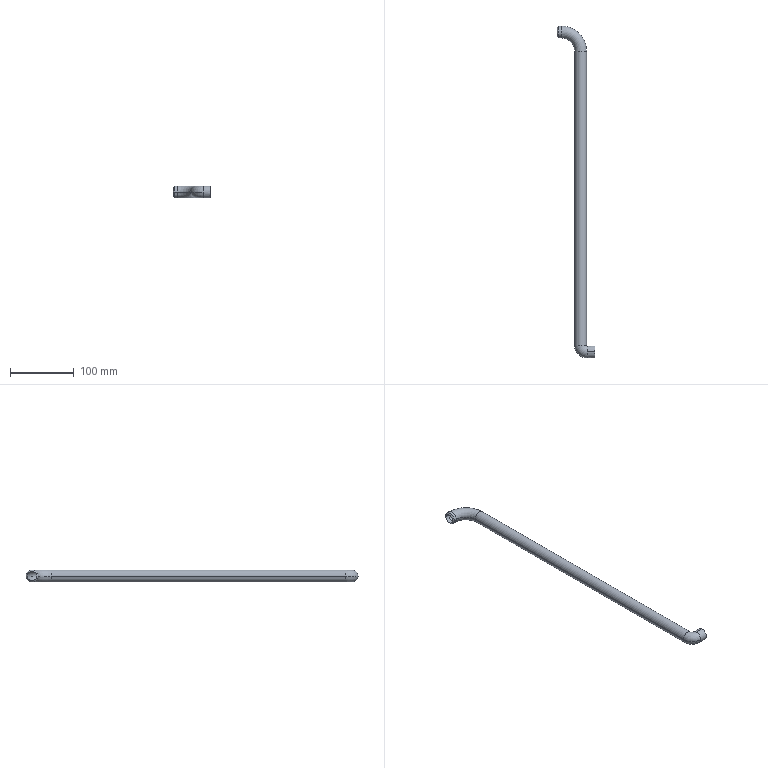Component | SolidWorks | PipeTwo-1 | 1 solid | 23 faces | box 59.27 x 519.6 x 18.77 mm | volume 54190 mm3 | cylinder 12 | torus 8 | cone 2 | plane 1 | commonest cylinder face diameters 15 x6 18.77 x6
STEP:
#1=COLOUR_RGB('',0.7922,0.8196,0.9333);
#2=FILL_AREA_STYLE_COLOUR('',#1);
#3=FILL_AREA_STYLE('',(#2));
#4=SURFACE_STYLE_FILL_AREA(#3);
#5=SURFACE_SIDE_STYLE('',(#4));
#6=SURFACE_STYLE_USAGE(.BOTH.,#5);
#7=PRESENTATION_STYLE_ASSIGNMENT((#6));
#8=CARTESIAN_POINT('',(24.858,12.574,4.921));
#9=VERTEX_POINT('',#8);
#10=CARTESIAN_POINT('',(25.448,12.574,4.921));
#11=VERTEX_POINT('',#10);
#12=CARTESIAN_POINT('',(25.153,12.574,4.921));
#13=DIRECTION('',(0.,-1.,0.));
#14=DIRECTION('',(0.,0.,1.));
#15=AXIS2_PLACEMENT_3D('',#12,#13,#14);
#16=CIRCLE('',#15,0.2953);
#17=EDGE_CURVE('',#9,#11,#16,.T.);
#18=ORIENTED_EDGE('',*,*,#17,.F.);
#19=CARTESIAN_POINT('',(25.547,11.885,4.921));
#20=VERTEX_POINT('',#19);
#21=CARTESIAN_POINT('',(25.547,12.574,4.921));
#22=DIRECTION('',(0.,0.,1.));
#23=DIRECTION('',(1.,0.,-0.));
#24=AXIS2_PLACEMENT_3D('',#21,#22,#23);
#25=CIRCLE('',#24,0.689);
#26=EDGE_CURVE('',#9,#20,#25,.T.);
#27=ORIENTED_EDGE('',*,*,#26,.T.);
#28=CARTESIAN_POINT('',(25.547,12.18,4.626));
#29=VERTEX_POINT('',#28);
#30=CARTESIAN_POINT('',(25.547,12.18,4.921));
#31=DIRECTION('',(1.,0.,-0.));
#32=DIRECTION('',(0.,0.,1.));
#33=AXIS2_PLACEMENT_3D('',#30,#31,#32);
#34=CIRCLE('',#33,0.2953);
#35=EDGE_CURVE('',#20,#29,#34,.T.);
#36=ORIENTED_EDGE('',*,*,#35,.T.);
#37=CARTESIAN_POINT('',(25.547,12.475,4.921));
#38=VERTEX_POINT('',#37);
#39=CARTESIAN_POINT('',(25.547,12.18,4.921));
#40=DIRECTION('',(1.,0.,-0.));
#41=DIRECTION('',(0.,0.,1.));
#42=AXIS2_PLACEMENT_3D('',#39,#40,#41);
#43=CIRCLE('',#42,0.2953);
#44=EDGE_CURVE('',#29,#38,#43,.T.);
#45=ORIENTED_EDGE('',*,*,#44,.T.);
#46=CARTESIAN_POINT('',(25.547,12.574,4.921));
#47=DIRECTION('',(0.,0.,1.));
#48=DIRECTION('',(1.,0.,0.));
#49=AXIS2_PLACEMENT_3D('',#46,#47,#48);
#50=CIRCLE('',#49,0.09843);
#51=EDGE_CURVE('',#11,#38,#50,.T.);
#52=ORIENTED_EDGE('',*,*,#51,.F.);
#53=EDGE_LOOP('',(#18,#27,#36,#45,#52));
#54=FACE_OUTER_BOUND('',#53,.T.);
#55=CARTESIAN_POINT('',(25.547,12.574,4.921));
#56=DIRECTION('',(0.,0.,1.));
#57=DIRECTION('',(1.,0.,-0.));
#58=AXIS2_PLACEMENT_3D('',#55,#56,#57);
#59=TOROIDAL_SURFACE('',#58,0.3937,0.2953);
#60=ADVANCED_FACE('',(#54),#59,.F.);
#61=CARTESIAN_POINT('',(23.972,32.193,4.921));
#62=VERTEX_POINT('',#61);
#63=CARTESIAN_POINT('',(23.972,31.602,4.921));
#64=VERTEX_POINT('',#63);
#65=CARTESIAN_POINT('',(23.972,31.898,4.921));
#66=DIRECTION('',(1.,0.,-0.));
#67=DIRECTION('',(0.,0.,1.));
#68=AXIS2_PLACEMENT_3D('',#65,#66,#67);
#69=CIRCLE('',#68,0.2953);
#70=EDGE_CURVE('',#62,#64,#69,.T.);
#71=ORIENTED_EDGE('',*,*,#70,.F.);
#72=CARTESIAN_POINT('',(25.448,30.717,4.921));
#73=VERTEX_POINT('',#72);
#74=CARTESIAN_POINT('',(23.972,30.717,4.921));
#75=DIRECTION('',(-0.,-0.,-1.));
#76=DIRECTION('',(-1.,0.,0.));
#77=AXIS2_PLACEMENT_3D('',#74,#75,#76);
#78=CIRCLE('',#77,1.476);
#79=EDGE_CURVE('',#62,#73,#78,.T.);
#80=ORIENTED_EDGE('',*,*,#79,.T.);
#81=CARTESIAN_POINT('',(24.858,30.717,4.921));
#82=VERTEX_POINT('',#81);
#83=CARTESIAN_POINT('',(25.153,30.717,4.921));
#84=DIRECTION('',(0.,-1.,0.));
#85=DIRECTION('',(0.,0.,1.));
#86=AXIS2_PLACEMENT_3D('',#83,#84,#85);
#87=CIRCLE('',#86,0.2953);
#88=EDGE_CURVE('',#73,#82,#87,.T.);
#89=ORIENTED_EDGE('',*,*,#88,.T.);
#90=CARTESIAN_POINT('',(23.972,30.717,4.921));
#91=DIRECTION('',(-0.,-0.,-1.));
#92=DIRECTION('',(-1.,0.,0.));
#93=AXIS2_PLACEMENT_3D('',#90,#91,#92);
#94=CIRCLE('',#93,0.8858);
#95=EDGE_CURVE('',#64,#82,#94,.T.);
#96=ORIENTED_EDGE('',*,*,#95,.F.);
#97=EDGE_LOOP('',(#71,#80,#89,#96));
#98=FACE_OUTER_BOUND('',#97,.T.);
#99=CARTESIAN_POINT('',(23.972,30.717,4.921));
#100=DIRECTION('',(-0.,-0.,-1.));
#101=DIRECTION('',(-1.,-0.,0.));
#102=AXIS2_PLACEMENT_3D('',#99,#100,#101);
#103=TOROIDAL_SURFACE('',#102,1.181,0.2953);
#104=ADVANCED_FACE('',(#98),#103,.F.);
#105=CARTESIAN_POINT('',(24.784,12.574,4.921));
#106=VERTEX_POINT('',#105);
#107=CARTESIAN_POINT('',(25.523,12.574,4.921));
#108=VERTEX_POINT('',#107);
#109=CARTESIAN_POINT('',(25.153,12.574,4.921));
#110=DIRECTION('',(-0.,1.,-0.));
#111=DIRECTION('',(0.,0.,1.));
#112=AXIS2_PLACEMENT_3D('',#109,#110,#111);
#113=CIRCLE('',#112,0.3695);
#114=EDGE_CURVE('',#106,#108,#113,.T.);
#115=ORIENTED_EDGE('',*,*,#114,.F.);
#116=CARTESIAN_POINT('',(25.547,11.81,4.921));
#117=VERTEX_POINT('',#116);
#118=CARTESIAN_POINT('',(25.547,12.574,4.921));
#119=DIRECTION('',(0.,0.,1.));
#120=DIRECTION('',(1.,0.,-0.));
#121=AXIS2_PLACEMENT_3D('',#118,#119,#120);
#122=CIRCLE('',#121,0.7632);
#123=EDGE_CURVE('',#106,#117,#122,.T.);
#124=ORIENTED_EDGE('',*,*,#123,.T.);
#125=CARTESIAN_POINT('',(25.547,12.18,5.291));
#126=VERTEX_POINT('',#125);
#127=CARTESIAN_POINT('',(25.547,12.18,4.921));
#128=DIRECTION('',(-1.,-0.,0.));
#129=DIRECTION('',(0.,0.,1.));
#130=AXIS2_PLACEMENT_3D('',#127,#128,#129);
#131=CIRCLE('',#130,0.3695);
#132=EDGE_CURVE('',#117,#126,#131,.T.);
#133=ORIENTED_EDGE('',*,*,#132,.T.);
#134=CARTESIAN_POINT('',(25.547,12.549,4.921));
#135=VERTEX_POINT('',#134);
#136=CARTESIAN_POINT('',(25.547,12.18,4.921));
#137=DIRECTION('',(-1.,-0.,0.));
#138=DIRECTION('',(0.,0.,1.));
#139=AXIS2_PLACEMENT_3D('',#136,#137,#138);
#140=CIRCLE('',#139,0.3695);
#141=EDGE_CURVE('',#126,#135,#140,.T.);
#142=ORIENTED_EDGE('',*,*,#141,.T.);
#143=CARTESIAN_POINT('',(25.547,12.574,4.921));
#144=DIRECTION('',(0.,0.,1.));
#145=DIRECTION('',(1.,0.,0.));
#146=AXIS2_PLACEMENT_3D('',#143,#144,#145);
#147=CIRCLE('',#146,0.02421);
#148=EDGE_CURVE('',#108,#135,#147,.T.);
#149=ORIENTED_EDGE('',*,*,#148,.F.);
#150=EDGE_LOOP('',(#115,#124,#133,#142,#149));
#151=FACE_OUTER_BOUND('',#150,.T.);
#152=CARTESIAN_POINT('',(25.547,12.574,4.921));
#153=DIRECTION('',(0.,0.,1.));
#154=DIRECTION('',(1.,0.,-0.));
#155=AXIS2_PLACEMENT_3D('',#152,#153,#154);
#156=TOROIDAL_SURFACE('',#155,0.3937,0.3695);
#157=ADVANCED_FACE('',(#151),#156,.T.);
#158=CARTESIAN_POINT('',(23.972,32.267,4.921));
#159=VERTEX_POINT('',#158);
#160=CARTESIAN_POINT('',(23.972,31.528,4.921));
#161=VERTEX_POINT('',#160);
#162=CARTESIAN_POINT('',(23.972,31.898,4.921));
#163=DIRECTION('',(-1.,-0.,0.));
#164=DIRECTION('',(0.,0.,1.));
#165=AXIS2_PLACEMENT_3D('',#162,#163,#164);
#166=CIRCLE('',#165,0.3695);
#167=EDGE_CURVE('',#159,#161,#166,.T.);
#168=ORIENTED_EDGE('',*,*,#167,.F.);
#169=CARTESIAN_POINT('',(25.523,30.717,4.921));
#170=VERTEX_POINT('',#169);
#171=CARTESIAN_POINT('',(23.972,30.717,4.921));
#172=DIRECTION('',(-0.,-0.,-1.));
#173=DIRECTION('',(-1.,0.,0.));
#174=AXIS2_PLACEMENT_3D('',#171,#172,#173);
#175=CIRCLE('',#174,1.551);
#176=EDGE_CURVE('',#159,#170,#175,.T.);
#177=ORIENTED_EDGE('',*,*,#176,.T.);
#178=CARTESIAN_POINT('',(24.784,30.717,4.921));
#179=VERTEX_POINT('',#178);
#180=CARTESIAN_POINT('',(25.153,30.717,4.921));
#181=DIRECTION('',(-0.,1.,-0.));
#182=DIRECTION('',(0.,0.,1.));
#183=AXIS2_PLACEMENT_3D('',#180,#181,#182);
#184=CIRCLE('',#183,0.3695);
#185=EDGE_CURVE('',#170,#179,#184,.T.);
#186=ORIENTED_EDGE('',*,*,#185,.T.);
#187=CARTESIAN_POINT('',(23.972,30.717,4.921));
#188=DIRECTION('',(-0.,-0.,-1.));
#189=DIRECTION('',(-1.,0.,0.));
#190=AXIS2_PLACEMENT_3D('',#187,#188,#189);
#191=CIRCLE('',#190,0.8116);
#192=EDGE_CURVE('',#161,#179,#191,.T.);
#193=ORIENTED_EDGE('',*,*,#192,.F.);
#194=EDGE_LOOP('',(#168,#177,#186,#193));
#195=FACE_OUTER_BOUND('',#194,.T.);
#196=CARTESIAN_POINT('',(23.972,30.717,4.921));
#197=DIRECTION('',(-0.,-0.,-1.));
#198=DIRECTION('',(-1.,-0.,0.));
#199=AXIS2_PLACEMENT_3D('',#196,#197,#198);
#200=TOROIDAL_SURFACE('',#199,1.181,0.3695);
#201=ADVANCED_FACE('',(#195),#200,.T.);
#202=CARTESIAN_POINT('',(23.701,32.193,4.921));
#203=VERTEX_POINT('',#202);
#204=CARTESIAN_POINT('',(23.701,31.602,4.921));
#205=VERTEX_POINT('',#204);
#206=CARTESIAN_POINT('',(23.701,31.898,4.921));
#207=DIRECTION('',(-1.,-0.,0.));
#208=DIRECTION('',(0.,-1.,0.));
#209=AXIS2_PLACEMENT_3D('',#206,#207,#208);
#210=CIRCLE('',#209,0.2953);
#211=EDGE_CURVE('',#203,#205,#210,.T.);
#212=ORIENTED_EDGE('',*,*,#211,.F.);
#213=CARTESIAN_POINT('',(23.775,32.267,4.921));
#214=VERTEX_POINT('',#213);
#215=CARTESIAN_POINT('',(23.578,32.07,4.921));
#216=DIRECTION('',(0.7071,0.7071,-0.));
#217=VECTOR('',#216,39.37);
#218=LINE('',#215,#217);
#219=EDGE_CURVE('',#203,#214,#218,.T.);
#220=ORIENTED_EDGE('',*,*,#219,.T.);
#221=CARTESIAN_POINT('',(23.775,31.528,4.921));
#222=VERTEX_POINT('',#221);
#223=CARTESIAN_POINT('',(23.775,31.898,4.921));
#224=DIRECTION('',(1.,0.,-0.));
#225=DIRECTION('',(0.,1.,0.));
#226=AXIS2_PLACEMENT_3D('',#223,#224,#225);
#227=CIRCLE('',#226,0.3695);
#228=EDGE_CURVE('',#222,#214,#227,.T.);
#229=ORIENTED_EDGE('',*,*,#228,.F.);
#230=CARTESIAN_POINT('',(23.578,31.725,4.921));
#231=DIRECTION('',(0.7071,-0.7071,-0.));
#232=VECTOR('',#231,39.37);
#233=LINE('',#230,#232);
#234=EDGE_CURVE('',#205,#222,#233,.T.);
#235=ORIENTED_EDGE('',*,*,#234,.F.);
#236=EDGE_LOOP('',(#212,#220,#229,#235));
#237=FACE_OUTER_BOUND('',#236,.T.);
#238=CARTESIAN_POINT('',(23.578,31.898,4.921));
#239=DIRECTION('',(1.,0.,-0.));
#240=DIRECTION('',(0.,-1.,0.));
#241=AXIS2_PLACEMENT_3D('',#238,#239,#240);
#242=CONICAL_SURFACE('',#241,0.1726,0.7854);
#243=ADVANCED_FACE('',(#237),#242,.T.);
#244=CARTESIAN_POINT('',(25.547,12.18,5.217));
#245=VERTEX_POINT('',#244);
#246=CARTESIAN_POINT('',(25.547,12.18,4.921));
#247=DIRECTION('',(1.,0.,-0.));
#248=DIRECTION('',(0.,0.,1.));
#249=AXIS2_PLACEMENT_3D('',#246,#247,#248);
#250=CIRCLE('',#249,0.2953);
#251=EDGE_CURVE('',#245,#20,#250,.T.);
#252=ORIENTED_EDGE('',*,*,#251,.F.);
#253=CARTESIAN_POINT('',(26.034,12.18,5.217));
#254=VERTEX_POINT('',#253);
#255=CARTESIAN_POINT('',(25.547,12.18,5.217));
#256=DIRECTION('',(1.,0.,-0.));
#257=VECTOR('',#256,39.37);
#258=LINE('',#255,#257);
#259=EDGE_CURVE('',#245,#254,#258,.T.);
#260=ORIENTED_EDGE('',*,*,#259,.T.);
#261=CARTESIAN_POINT('',(26.034,12.18,4.626));
#262=VERTEX_POINT('',#261);
#263=CARTESIAN_POINT('',(26.034,12.18,4.921));
#264=DIRECTION('',(1.,0.,-0.));
#265=DIRECTION('',(0.,0.,1.));
#266=AXIS2_PLACEMENT_3D('',#263,#264,#265);
#267=CIRCLE('',#266,0.2953);
#268=EDGE_CURVE('',#254,#262,#267,.T.);
#269=ORIENTED_EDGE('',*,*,#268,.T.);
#270=CARTESIAN_POINT('',(25.547,12.18,4.626));
#271=DIRECTION('',(1.,0.,-0.));
#272=VECTOR('',#271,39.37);
#273=LINE('',#270,#272);
#274=EDGE_CURVE('',#29,#262,#273,.T.);
#275=ORIENTED_EDGE('',*,*,#274,.F.);
#276=ORIENTED_EDGE('',*,*,#35,.F.);
#277=EDGE_LOOP('',(#252,#260,#269,#275,#276));
#278=FACE_OUTER_BOUND('',#277,.T.);
#279=CARTESIAN_POINT('',(25.547,12.18,4.921));
#280=DIRECTION('',(1.,0.,-0.));
#281=DIRECTION('',(0.,0.,-1.));
#282=AXIS2_PLACEMENT_3D('',#279,#280,#281);
#283=CYLINDRICAL_SURFACE('',#282,0.2953);
#284=ADVANCED_FACE('',(#278),#283,.F.);
#285=ORIENTED_EDGE('',*,*,#88,.F.);
#286=CARTESIAN_POINT('',(25.448,30.717,4.921));
#287=DIRECTION('',(0.,-1.,0.));
#288=VECTOR('',#287,39.37);
#289=LINE('',#286,#288);
#290=EDGE_CURVE('',#73,#11,#289,.T.);
#291=ORIENTED_EDGE('',*,*,#290,.T.);
#292=CARTESIAN_POINT('',(25.153,12.574,4.921));
#293=DIRECTION('',(0.,-1.,0.));
#294=DIRECTION('',(0.,0.,1.));
#295=AXIS2_PLACEMENT_3D('',#292,#293,#294);
#296=CIRCLE('',#295,0.2953);
#297=EDGE_CURVE('',#11,#9,#296,.T.);
#298=ORIENTED_EDGE('',*,*,#297,.T.);
#299=CARTESIAN_POINT('',(24.858,30.717,4.921));
#300=DIRECTION('',(0.,-1.,0.));
#301=VECTOR('',#300,39.37);
#302=LINE('',#299,#301);
#303=EDGE_CURVE('',#82,#9,#302,.T.);
#304=ORIENTED_EDGE('',*,*,#303,.F.);
#305=EDGE_LOOP('',(#285,#291,#298,#304));
#306=FACE_OUTER_BOUND('',#305,.T.);
#307=CARTESIAN_POINT('',(25.153,30.717,4.921));
#308=DIRECTION('',(0.,-1.,0.));
#309=DIRECTION('',(-1.,0.,0.));
#310=AXIS2_PLACEMENT_3D('',#307,#308,#309);
#311=CYLINDRICAL_SURFACE('',#310,0.2953);
#312=ADVANCED_FACE('',(#306),#311,.F.);
#313=CARTESIAN_POINT('',(23.701,31.898,4.921));
#314=DIRECTION('',(-1.,-0.,0.));
#315=DIRECTION('',(0.,-1.,0.));
#316=AXIS2_PLACEMENT_3D('',#313,#314,#315);
#317=CIRCLE('',#316,0.2953);
#318=EDGE_CURVE('',#205,#203,#317,.T.);
#319=ORIENTED_EDGE('',*,*,#318,.T.);
#320=CARTESIAN_POINT('',(23.578,32.193,4.921));
#321=DIRECTION('',(1.,0.,-0.));
#322=VECTOR('',#321,39.37);
#323=LINE('',#320,#322);
#324=EDGE_CURVE('',#203,#62,#323,.T.);
#325=ORIENTED_EDGE('',*,*,#324,.T.);
#326=ORIENTED_EDGE('',*,*,#70,.T.);
#327=CARTESIAN_POINT('',(23.578,31.602,4.921));
#328=DIRECTION('',(1.,0.,-0.));
#329=VECTOR('',#328,39.37);
#330=LINE('',#327,#329);
#331=EDGE_CURVE('',#205,#64,#330,.T.);
#332=ORIENTED_EDGE('',*,*,#331,.F.);
#333=EDGE_LOOP('',(#319,#325,#326,#332));
#334=FACE_OUTER_BOUND('',#333,.T.);
#335=CARTESIAN_POINT('',(23.578,31.898,4.921));
#336=DIRECTION('',(1.,0.,-0.));
#337=DIRECTION('',(0.,-1.,0.));
#338=AXIS2_PLACEMENT_3D('',#335,#336,#337);
#339=CYLINDRICAL_SURFACE('',#338,0.2953);
#340=ADVANCED_FACE('',(#334),#339,.F.);
#341=ORIENTED_EDGE('',*,*,#141,.F.);
#342=CARTESIAN_POINT('',(26.034,12.18,5.291));
#343=VERTEX_POINT('',#342);
#344=CARTESIAN_POINT('',(25.547,12.18,5.291));
#345=DIRECTION('',(1.,0.,-0.));
#346=VECTOR('',#345,39.37);
#347=LINE('',#344,#346);
#348=EDGE_CURVE('',#126,#343,#347,.T.);
#349=ORIENTED_EDGE('',*,*,#348,.T.);
#350=CARTESIAN_POINT('',(26.034,12.18,4.552));
#351=VERTEX_POINT('',#350);
#352=CARTESIAN_POINT('',(26.034,12.18,4.921));
#353=DIRECTION('',(-1.,-0.,0.));
#354=DIRECTION('',(0.,0.,1.));
#355=AXIS2_PLACEMENT_3D('',#352,#353,#354);
#356=CIRCLE('',#355,0.3695);
#357=EDGE_CURVE('',#343,#351,#356,.T.);
#358=ORIENTED_EDGE('',*,*,#357,.T.);
#359=CARTESIAN_POINT('',(25.547,12.18,4.552));
#360=VERTEX_POINT('',#359);
#361=CARTESIAN_POINT('',(25.547,12.18,4.552));
#362=DIRECTION('',(1.,0.,-0.));
#363=VECTOR('',#362,39.37);
#364=LINE('',#361,#363);
#365=EDGE_CURVE('',#360,#351,#364,.T.);
#366=ORIENTED_EDGE('',*,*,#365,.F.);
#367=CARTESIAN_POINT('',(25.547,12.18,4.921));
#368=DIRECTION('',(-1.,-0.,0.));
#369=DIRECTION('',(0.,0.,1.));
#370=AXIS2_PLACEMENT_3D('',#367,#368,#369);
#371=CIRCLE('',#370,0.3695);
#372=EDGE_CURVE('',#135,#360,#371,.T.);
#373=ORIENTED_EDGE('',*,*,#372,.F.);
#374=EDGE_LOOP('',(#341,#349,#358,#366,#373));
#375=FACE_OUTER_BOUND('',#374,.T.);
#376=CARTESIAN_POINT('',(25.547,12.18,4.921));
#377=DIRECTION('',(1.,0.,-0.));
#378=DIRECTION('',(0.,0.,-1.));
#379=AXIS2_PLACEMENT_3D('',#376,#377,#378);
#380=CYLINDRICAL_SURFACE('',#379,0.3695);
#381=ADVANCED_FACE('',(#375),#380,.T.);
#382=ORIENTED_EDGE('',*,*,#185,.F.);
#383=CARTESIAN_POINT('',(25.523,30.717,4.921));
#384=DIRECTION('',(0.,-1.,0.));
#385=VECTOR('',#384,39.37);
#386=LINE('',#383,#385);
#387=EDGE_CURVE('',#170,#108,#386,.T.);
#388=ORIENTED_EDGE('',*,*,#387,.T.);
#389=CARTESIAN_POINT('',(25.153,12.574,4.921));
#390=DIRECTION('',(-0.,1.,-0.));
#391=DIRECTION('',(0.,0.,1.));
#392=AXIS2_PLACEMENT_3D('',#389,#390,#391);
#393=CIRCLE('',#392,0.3695);
#394=EDGE_CURVE('',#108,#106,#393,.T.);
#395=ORIENTED_EDGE('',*,*,#394,.T.);
#396=CARTESIAN_POINT('',(24.784,30.717,4.921));
#397=DIRECTION('',(0.,-1.,0.));
#398=VECTOR('',#397,39.37);
#399=LINE('',#396,#398);
#400=EDGE_CURVE('',#179,#106,#399,.T.);
#401=ORIENTED_EDGE('',*,*,#400,.F.);
#402=EDGE_LOOP('',(#382,#388,#395,#401));
#403=FACE_OUTER_BOUND('',#402,.T.);
#404=CARTESIAN_POINT('',(25.153,30.717,4.921));
#405=DIRECTION('',(0.,-1.,0.));
#406=DIRECTION('',(-1.,0.,0.));
#407=AXIS2_PLACEMENT_3D('',#404,#405,#406);
#408=CYLINDRICAL_SURFACE('',#407,0.3695);
#409=ADVANCED_FACE('',(#403),#408,.T.);
#410=ORIENTED_EDGE('',*,*,#228,.T.);
#411=CARTESIAN_POINT('',(23.578,32.267,4.921));
#412=DIRECTION('',(1.,0.,-0.));
#413=VECTOR('',#412,39.37);
#414=LINE('',#411,#413);
#415=EDGE_CURVE('',#214,#159,#414,.T.);
#416=ORIENTED_EDGE('',*,*,#415,.T.);
#417=ORIENTED_EDGE('',*,*,#167,.T.);
#418=CARTESIAN_POINT('',(23.578,31.528,4.921));
#419=DIRECTION('',(1.,0.,-0.));
#420=VECTOR('',#419,39.37);
#421=LINE('',#418,#420);
#422=EDGE_CURVE('',#222,#161,#421,.T.);
#423=ORIENTED_EDGE('',*,*,#422,.F.);
#424=EDGE_LOOP('',(#410,#416,#417,#423));
#425=FACE_OUTER_BOUND('',#424,.T.);
#426=CARTESIAN_POINT('',(23.578,31.898,4.921));
#427=DIRECTION('',(1.,0.,-0.));
#428=DIRECTION('',(0.,-1.,0.));
#429=AXIS2_PLACEMENT_3D('',#426,#427,#428);
#430=CYLINDRICAL_SURFACE('',#429,0.3695);
#431=ADVANCED_FACE('',(#425),#430,.T.);
#432=ORIENTED_EDGE('',*,*,#259,.F.);
#433=CARTESIAN_POINT('',(25.547,12.18,4.921));
#434=DIRECTION('',(1.,0.,-0.));
#435=DIRECTION('',(0.,0.,1.));
#436=AXIS2_PLACEMENT_3D('',#433,#434,#435);
#437=CIRCLE('',#436,0.2953);
#438=EDGE_CURVE('',#38,#245,#437,.T.);
#439=ORIENTED_EDGE('',*,*,#438,.F.);
#440=ORIENTED_EDGE('',*,*,#44,.F.);
#441=ORIENTED_EDGE('',*,*,#274,.T.);
#442=CARTESIAN_POINT('',(26.034,12.18,4.921));
#443=DIRECTION('',(1.,0.,-0.));
#444=DIRECTION('',(0.,0.,1.));
#445=AXIS2_PLACEMENT_3D('',#442,#443,#444);
#446=CIRCLE('',#445,0.2953);
#447=EDGE_CURVE('',#262,#254,#446,.T.);
#448=ORIENTED_EDGE('',*,*,#447,.T.);
#449=EDGE_LOOP('',(#432,#439,#440,#441,#448));
#450=FACE_OUTER_BOUND('',#449,.T.);
#451=CARTESIAN_POINT('',(25.547,12.18,4.921));
#452=DIRECTION('',(1.,0.,-0.));
#453=DIRECTION('',(0.,0.,-1.));
#454=AXIS2_PLACEMENT_3D('',#451,#452,#453);
#455=CYLINDRICAL_SURFACE('',#454,0.2953);
#456=ADVANCED_FACE('',(#450),#455,.F.);
#457=ORIENTED_EDGE('',*,*,#26,.F.);
#458=ORIENTED_EDGE('',*,*,#297,.F.);
#459=ORIENTED_EDGE('',*,*,#51,.T.);
#460=ORIENTED_EDGE('',*,*,#438,.T.);
#461=ORIENTED_EDGE('',*,*,#251,.T.);
#462=EDGE_LOOP('',(#457,#458,#459,#460,#461));
#463=FACE_OUTER_BOUND('',#462,.T.);
#464=CARTESIAN_POINT('',(25.547,12.574,4.921));
#465=DIRECTION('',(0.,0.,1.));
#466=DIRECTION('',(1.,0.,-0.));
#467=AXIS2_PLACEMENT_3D('',#464,#465,#466);
#468=TOROIDAL_SURFACE('',#467,0.3937,0.2953);
#469=ADVANCED_FACE('',(#463),#468,.F.);
#470=ORIENTED_EDGE('',*,*,#290,.F.);
#471=CARTESIAN_POINT('',(25.153,30.717,4.921));
#472=DIRECTION('',(0.,-1.,0.));
#473=DIRECTION('',(0.,0.,1.));
#474=AXIS2_PLACEMENT_3D('',#471,#472,#473);
#475=CIRCLE('',#474,0.2953);
#476=EDGE_CURVE('',#82,#73,#475,.T.);
#477=ORIENTED_EDGE('',*,*,#476,.F.);
#478=ORIENTED_EDGE('',*,*,#303,.T.);
#479=ORIENTED_EDGE('',*,*,#17,.T.);
#480=EDGE_LOOP('',(#470,#477,#478,#479));
#481=FACE_OUTER_BOUND('',#480,.T.);
#482=CARTESIAN_POINT('',(25.153,30.717,4.921));
#483=DIRECTION('',(0.,-1.,0.));
#484=DIRECTION('',(-1.,0.,0.));
#485=AXIS2_PLACEMENT_3D('',#482,#483,#484);
#486=CYLINDRICAL_SURFACE('',#485,0.2953);
#487=ADVANCED_FACE('',(#481),#486,.F.);
#488=ORIENTED_EDGE('',*,*,#79,.F.);
#489=CARTESIAN_POINT('',(23.972,31.898,4.921));
#490=DIRECTION('',(1.,0.,-0.));
#491=DIRECTION('',(0.,0.,1.));
#492=AXIS2_PLACEMENT_3D('',#489,#490,#491);
#493=CIRCLE('',#492,0.2953);
#494=EDGE_CURVE('',#64,#62,#493,.T.);
#495=ORIENTED_EDGE('',*,*,#494,.F.);
#496=ORIENTED_EDGE('',*,*,#95,.T.);
#497=ORIENTED_EDGE('',*,*,#476,.T.);
#498=EDGE_LOOP('',(#488,#495,#496,#497));
#499=FACE_OUTER_BOUND('',#498,.T.);
#500=CARTESIAN_POINT('',(23.972,30.717,4.921));
#501=DIRECTION('',(-0.,-0.,-1.));
#502=DIRECTION('',(-1.,-0.,0.));
#503=AXIS2_PLACEMENT_3D('',#500,#501,#502);
#504=TOROIDAL_SURFACE('',#503,1.181,0.2953);
#505=ADVANCED_FACE('',(#499),#504,.F.);
#506=ORIENTED_EDGE('',*,*,#324,.F.);
#507=ORIENTED_EDGE('',*,*,#211,.T.);
#508=ORIENTED_EDGE('',*,*,#331,.T.);
#509=ORIENTED_EDGE('',*,*,#494,.T.);
#510=EDGE_LOOP('',(#506,#507,#508,#509));
#511=FACE_OUTER_BOUND('',#510,.T.);
#512=CARTESIAN_POINT('',(23.578,31.898,4.921));
#513=DIRECTION('',(1.,0.,-0.));
#514=DIRECTION('',(0.,-1.,0.));
#515=AXIS2_PLACEMENT_3D('',#512,#513,#514);
#516=CYLINDRICAL_SURFACE('',#515,0.2953);
#517=ADVANCED_FACE('',(#511),#516,.F.);
#518=ORIENTED_EDGE('',*,*,#447,.F.);
#519=ORIENTED_EDGE('',*,*,#268,.F.);
#520=EDGE_LOOP('',(#518,#519));
#521=FACE_BOUND('',#520,.T.);
#522=CARTESIAN_POINT('',(26.034,12.18,4.921));
#523=DIRECTION('',(-1.,-0.,0.));
#524=DIRECTION('',(0.,0.,1.));
#525=AXIS2_PLACEMENT_3D('',#522,#523,#524);
#526=CIRCLE('',#525,0.3695);
#527=EDGE_CURVE('',#351,#343,#526,.T.);
#528=ORIENTED_EDGE('',*,*,#527,.F.);
#529=ORIENTED_EDGE('',*,*,#357,.F.);
#530=EDGE_LOOP('',(#528,#529));
#531=FACE_OUTER_BOUND('',#530,.T.);
#532=CARTESIAN_POINT('',(26.034,12.18,4.921));
#533=DIRECTION('',(-1.,-0.,0.));
#534=DIRECTION('',(0.,0.,1.));
#535=AXIS2_PLACEMENT_3D('',#532,#533,#534);
#536=PLANE('',#535);
#537=ADVANCED_FACE('',(#521,#531),#536,.F.);
#538=ORIENTED_EDGE('',*,*,#348,.F.);
#539=ORIENTED_EDGE('',*,*,#132,.F.);
#540=CARTESIAN_POINT('',(25.547,12.18,4.921));
#541=DIRECTION('',(-1.,-0.,0.));
#542=DIRECTION('',(0.,0.,1.));
#543=AXIS2_PLACEMENT_3D('',#540,#541,#542);
#544=CIRCLE('',#543,0.3695);
#545=EDGE_CURVE('',#360,#117,#544,.T.);
#546=ORIENTED_EDGE('',*,*,#545,.F.);
#547=ORIENTED_EDGE('',*,*,#365,.T.);
#548=ORIENTED_EDGE('',*,*,#527,.T.);
#549=EDGE_LOOP('',(#538,#539,#546,#547,#548));
#550=FACE_OUTER_BOUND('',#549,.T.);
#551=CARTESIAN_POINT('',(25.547,12.18,4.921));
#552=DIRECTION('',(1.,0.,-0.));
#553=DIRECTION('',(0.,0.,-1.));
#554=AXIS2_PLACEMENT_3D('',#551,#552,#553);
#555=CYLINDRICAL_SURFACE('',#554,0.3695);
#556=ADVANCED_FACE('',(#550),#555,.T.);
#557=ORIENTED_EDGE('',*,*,#123,.F.);
#558=ORIENTED_EDGE('',*,*,#394,.F.);
#559=ORIENTED_EDGE('',*,*,#148,.T.);
#560=ORIENTED_EDGE('',*,*,#372,.T.);
#561=ORIENTED_EDGE('',*,*,#545,.T.);
#562=EDGE_LOOP('',(#557,#558,#559,#560,#561));
#563=FACE_OUTER_BOUND('',#562,.T.);
#564=CARTESIAN_POINT('',(25.547,12.574,4.921));
#565=DIRECTION('',(0.,0.,1.));
#566=DIRECTION('',(1.,0.,-0.));
#567=AXIS2_PLACEMENT_3D('',#564,#565,#566);
#568=TOROIDAL_SURFACE('',#567,0.3937,0.3695);
#569=ADVANCED_FACE('',(#563),#568,.T.);
#570=ORIENTED_EDGE('',*,*,#387,.F.);
#571=CARTESIAN_POINT('',(25.153,30.717,4.921));
#572=DIRECTION('',(-0.,1.,-0.));
#573=DIRECTION('',(0.,0.,1.));
#574=AXIS2_PLACEMENT_3D('',#571,#572,#573);
#575=CIRCLE('',#574,0.3695);
#576=EDGE_CURVE('',#179,#170,#575,.T.);
#577=ORIENTED_EDGE('',*,*,#576,.F.);
#578=ORIENTED_EDGE('',*,*,#400,.T.);
#579=ORIENTED_EDGE('',*,*,#114,.T.);
#580=EDGE_LOOP('',(#570,#577,#578,#579));
#581=FACE_OUTER_BOUND('',#580,.T.);
#582=CARTESIAN_POINT('',(25.153,30.717,4.921));
#583=DIRECTION('',(0.,-1.,0.));
#584=DIRECTION('',(-1.,0.,0.));
#585=AXIS2_PLACEMENT_3D('',#582,#583,#584);
#586=CYLINDRICAL_SURFACE('',#585,0.3695);
#587=ADVANCED_FACE('',(#581),#586,.T.);
#588=ORIENTED_EDGE('',*,*,#176,.F.);
#589=CARTESIAN_POINT('',(23.972,31.898,4.921));
#590=DIRECTION('',(-1.,-0.,0.));
#591=DIRECTION('',(0.,0.,1.));
#592=AXIS2_PLACEMENT_3D('',#589,#590,#591);
#593=CIRCLE('',#592,0.3695);
#594=EDGE_CURVE('',#161,#159,#593,.T.);
#595=ORIENTED_EDGE('',*,*,#594,.F.);
#596=ORIENTED_EDGE('',*,*,#192,.T.);
#597=ORIENTED_EDGE('',*,*,#576,.T.);
#598=EDGE_LOOP('',(#588,#595,#596,#597));
#599=FACE_OUTER_BOUND('',#598,.T.);
#600=CARTESIAN_POINT('',(23.972,30.717,4.921));
#601=DIRECTION('',(-0.,-0.,-1.));
#602=DIRECTION('',(-1.,-0.,0.));
#603=AXIS2_PLACEMENT_3D('',#600,#601,#602);
#604=TOROIDAL_SURFACE('',#603,1.181,0.3695);
#605=ADVANCED_FACE('',(#599),#604,.T.);
#606=ORIENTED_EDGE('',*,*,#415,.F.);
#607=CARTESIAN_POINT('',(23.775,31.898,4.921));
#608=DIRECTION('',(1.,0.,-0.));
#609=DIRECTION('',(0.,1.,0.));
#610=AXIS2_PLACEMENT_3D('',#607,#608,#609);
#611=CIRCLE('',#610,0.3695);
#612=EDGE_CURVE('',#214,#222,#611,.T.);
#613=ORIENTED_EDGE('',*,*,#612,.T.);
#614=ORIENTED_EDGE('',*,*,#422,.T.);
#615=ORIENTED_EDGE('',*,*,#594,.T.);
#616=EDGE_LOOP('',(#606,#613,#614,#615));
#617=FACE_OUTER_BOUND('',#616,.T.);
#618=CARTESIAN_POINT('',(23.578,31.898,4.921));
#619=DIRECTION('',(1.,0.,-0.));
#620=DIRECTION('',(0.,-1.,0.));
#621=AXIS2_PLACEMENT_3D('',#618,#619,#620);
#622=CYLINDRICAL_SURFACE('',#621,0.3695);
#623=ADVANCED_FACE('',(#617),#622,.T.);
#624=ORIENTED_EDGE('',*,*,#219,.F.);
#625=ORIENTED_EDGE('',*,*,#318,.F.);
#626=ORIENTED_EDGE('',*,*,#234,.T.);
#627=ORIENTED_EDGE('',*,*,#612,.F.);
#628=EDGE_LOOP('',(#624,#625,#626,#627));
#629=FACE_OUTER_BOUND('',#628,.T.);
#630=CARTESIAN_POINT('',(23.578,31.898,4.921));
#631=DIRECTION('',(1.,0.,-0.));
#632=DIRECTION('',(0.,-1.,0.));
#633=AXIS2_PLACEMENT_3D('',#630,#631,#632);
#634=CONICAL_SURFACE('',#633,0.1726,0.7854);
#635=ADVANCED_FACE('',(#629),#634,.T.);
#636=CLOSED_SHELL('',(#60,#104,#157,#201,#243,#284,#312,#340,#381,#409,#431,#456,#469,#487,#505,#517,#537,#556,#569,#587,#605,#623,#635));
#637=MANIFOLD_SOLID_BREP('',#636);
#638=STYLED_ITEM('',(#7),#637);
#639=PRESENTATION_LAYER_ASSIGNMENT('','',(#638));
#640=CARTESIAN_POINT('',(0.,0.,0.));
#641=DIRECTION('',(0.,0.,1.));
#642=DIRECTION('',(1.,0.,0.));
#643=AXIS2_PLACEMENT_3D('',#640,#641,#642);
#644=(LENGTH_UNIT()NAMED_UNIT(*)SI_UNIT($,.METRE.));
#645=LENGTH_MEASURE_WITH_UNIT(LENGTH_MEASURE(0.0254),#644);
#646=DIMENSIONAL_EXPONENTS(1.,0.,0.,0.,0.,0.,0.);
#647=(CONVERSION_BASED_UNIT('',#645)LENGTH_UNIT()NAMED_UNIT(#646));
#648=UNCERTAINTY_MEASURE_WITH_UNIT(LENGTH_MEASURE(0.00001),#647,'','');
#649=(NAMED_UNIT(*)PLANE_ANGLE_UNIT()SI_UNIT($,.RADIAN.));
#650=(NAMED_UNIT(*)SI_UNIT($,.STERADIAN.)SOLID_ANGLE_UNIT());
#651=(GEOMETRIC_REPRESENTATION_CONTEXT(3)GLOBAL_UNCERTAINTY_ASSIGNED_CONTEXT((#648))GLOBAL_UNIT_ASSIGNED_CONTEXT((#647,#649,#650))REPRESENTATION_CONTEXT('',''));
#652=ADVANCED_BREP_SHAPE_REPRESENTATION('',(#637,#643),#651);
#653=(LENGTH_UNIT()NAMED_UNIT(*)SI_UNIT($,.METRE.));
#654=LENGTH_MEASURE_WITH_UNIT(LENGTH_MEASURE(0.0254),#653);
#655=DIMENSIONAL_EXPONENTS(1.,0.,0.,0.,0.,0.,0.);
#656=(CONVERSION_BASED_UNIT('',#654)LENGTH_UNIT()NAMED_UNIT(#655));
#657=UNCERTAINTY_MEASURE_WITH_UNIT(LENGTH_MEASURE(0.00001),#656,'','');
#658=(NAMED_UNIT(*)PLANE_ANGLE_UNIT()SI_UNIT($,.RADIAN.));
#659=(NAMED_UNIT(*)SI_UNIT($,.STERADIAN.)SOLID_ANGLE_UNIT());
#660=(GEOMETRIC_REPRESENTATION_CONTEXT(3)GLOBAL_UNCERTAINTY_ASSIGNED_CONTEXT((#657))GLOBAL_UNIT_ASSIGNED_CONTEXT((#656,#658,#659))REPRESENTATION_CONTEXT('',''));
#661=MECHANICAL_DESIGN_GEOMETRIC_PRESENTATION_REPRESENTATION('',(#638),#660);